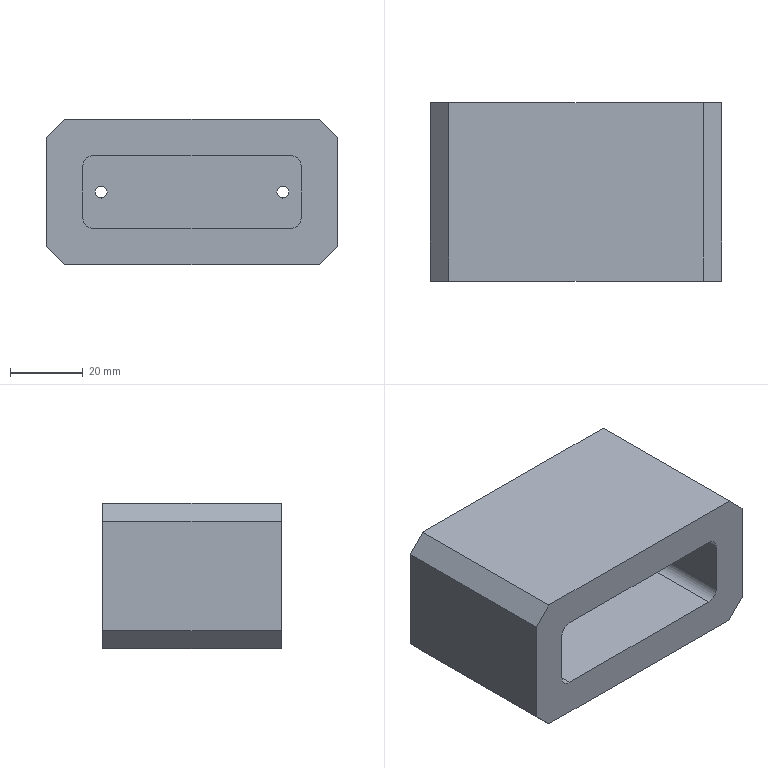CAM job | Mastercam | mm | 10 operations | part box 80 x 49 x 40
1. Facing | 24 - 100 平铣刀
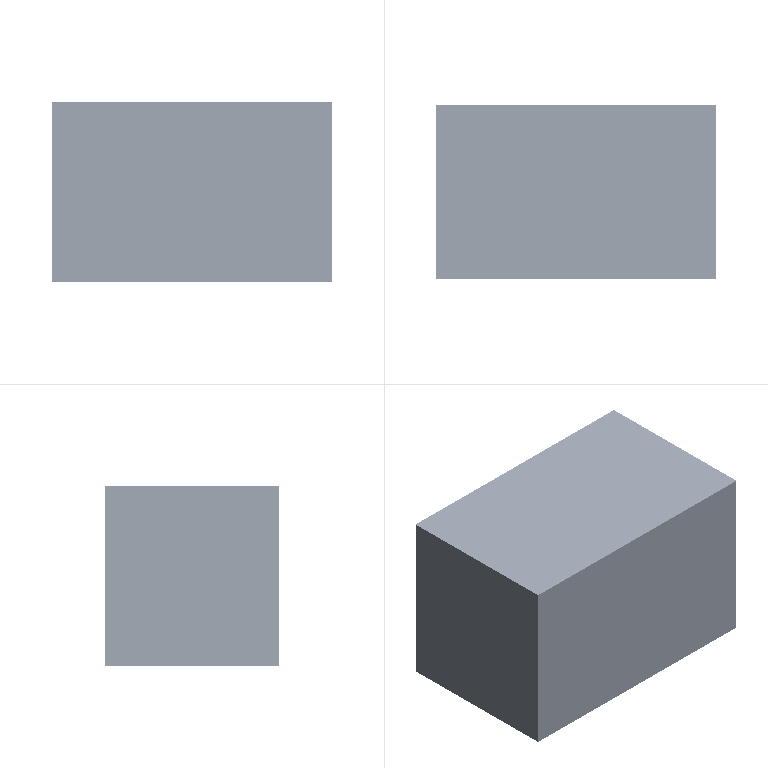2. 2D High Speed (2D Dynamic Mill) | 12 - 12 平铣刀
3. Contour (2D) | 12 - 12 平铣刀
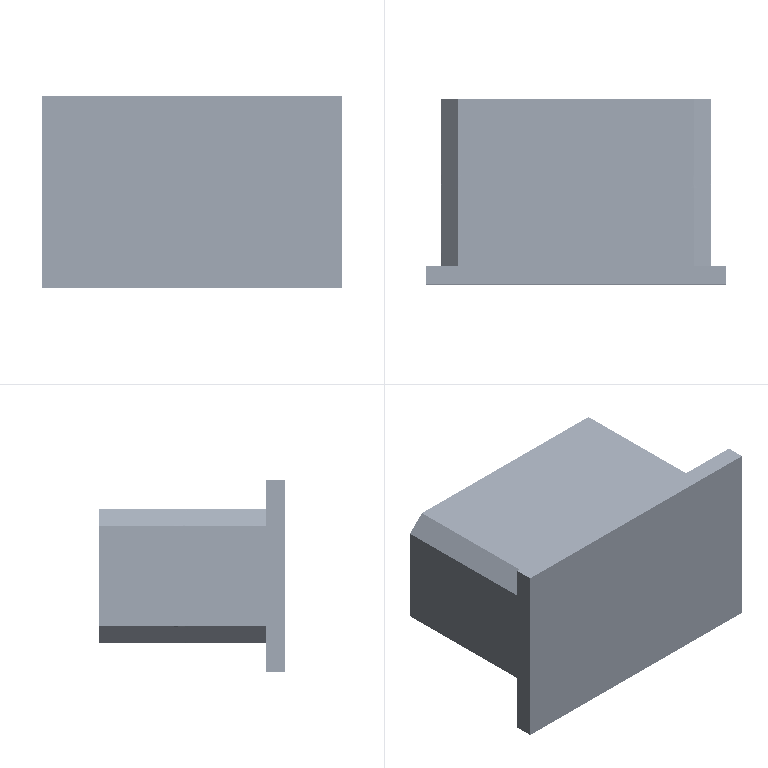4. Drill/Counterbore | 7 - 4 倒角刀
5. Contour (2D chamfer) | 7 - 4 倒角刀
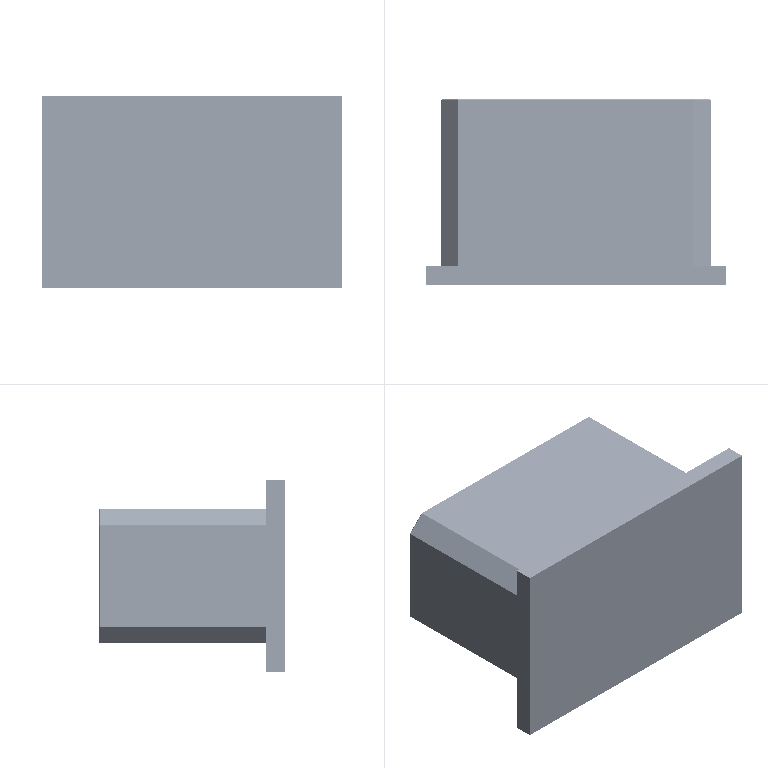6. Facing | 24 - 100 平铣刀
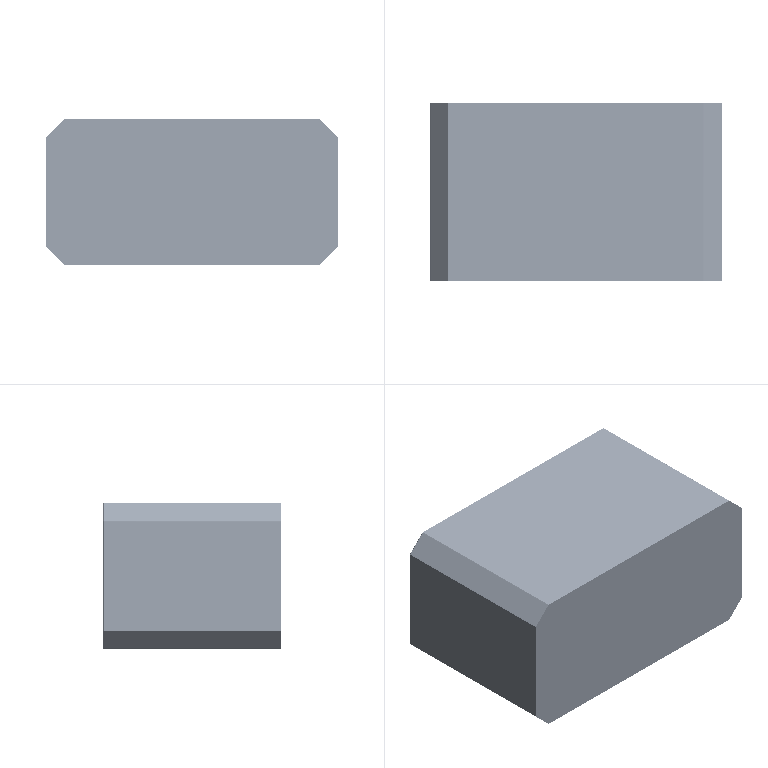7. Contour (Ramp) | 12 - 12 平铣刀
8. Contour (Remachining) | 6 - 6 平铣刀
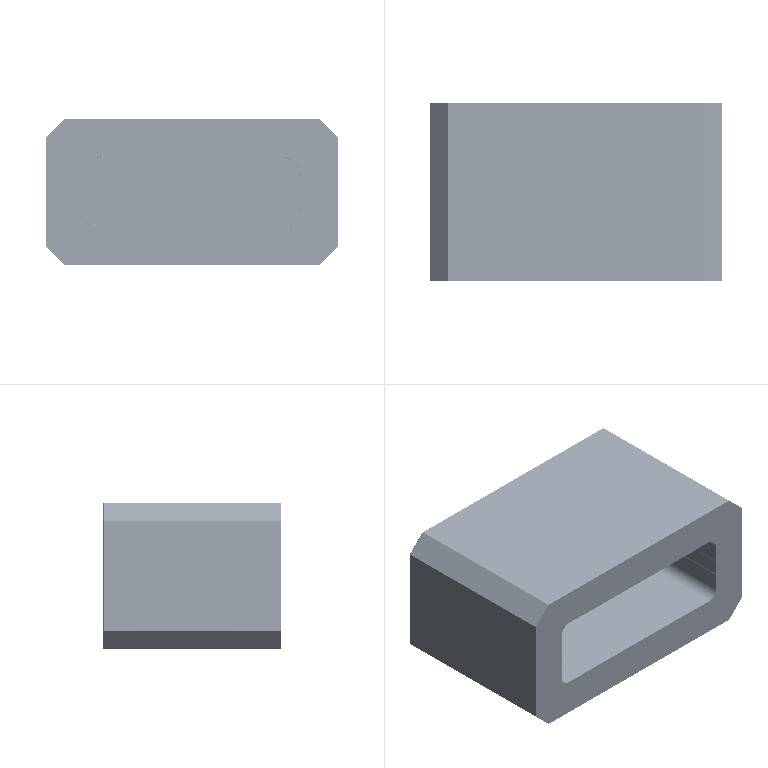9. Contour (2D) | 6 - 6 平铣刀
10. Contour (2D chamfer) | 7 - 4 倒角刀